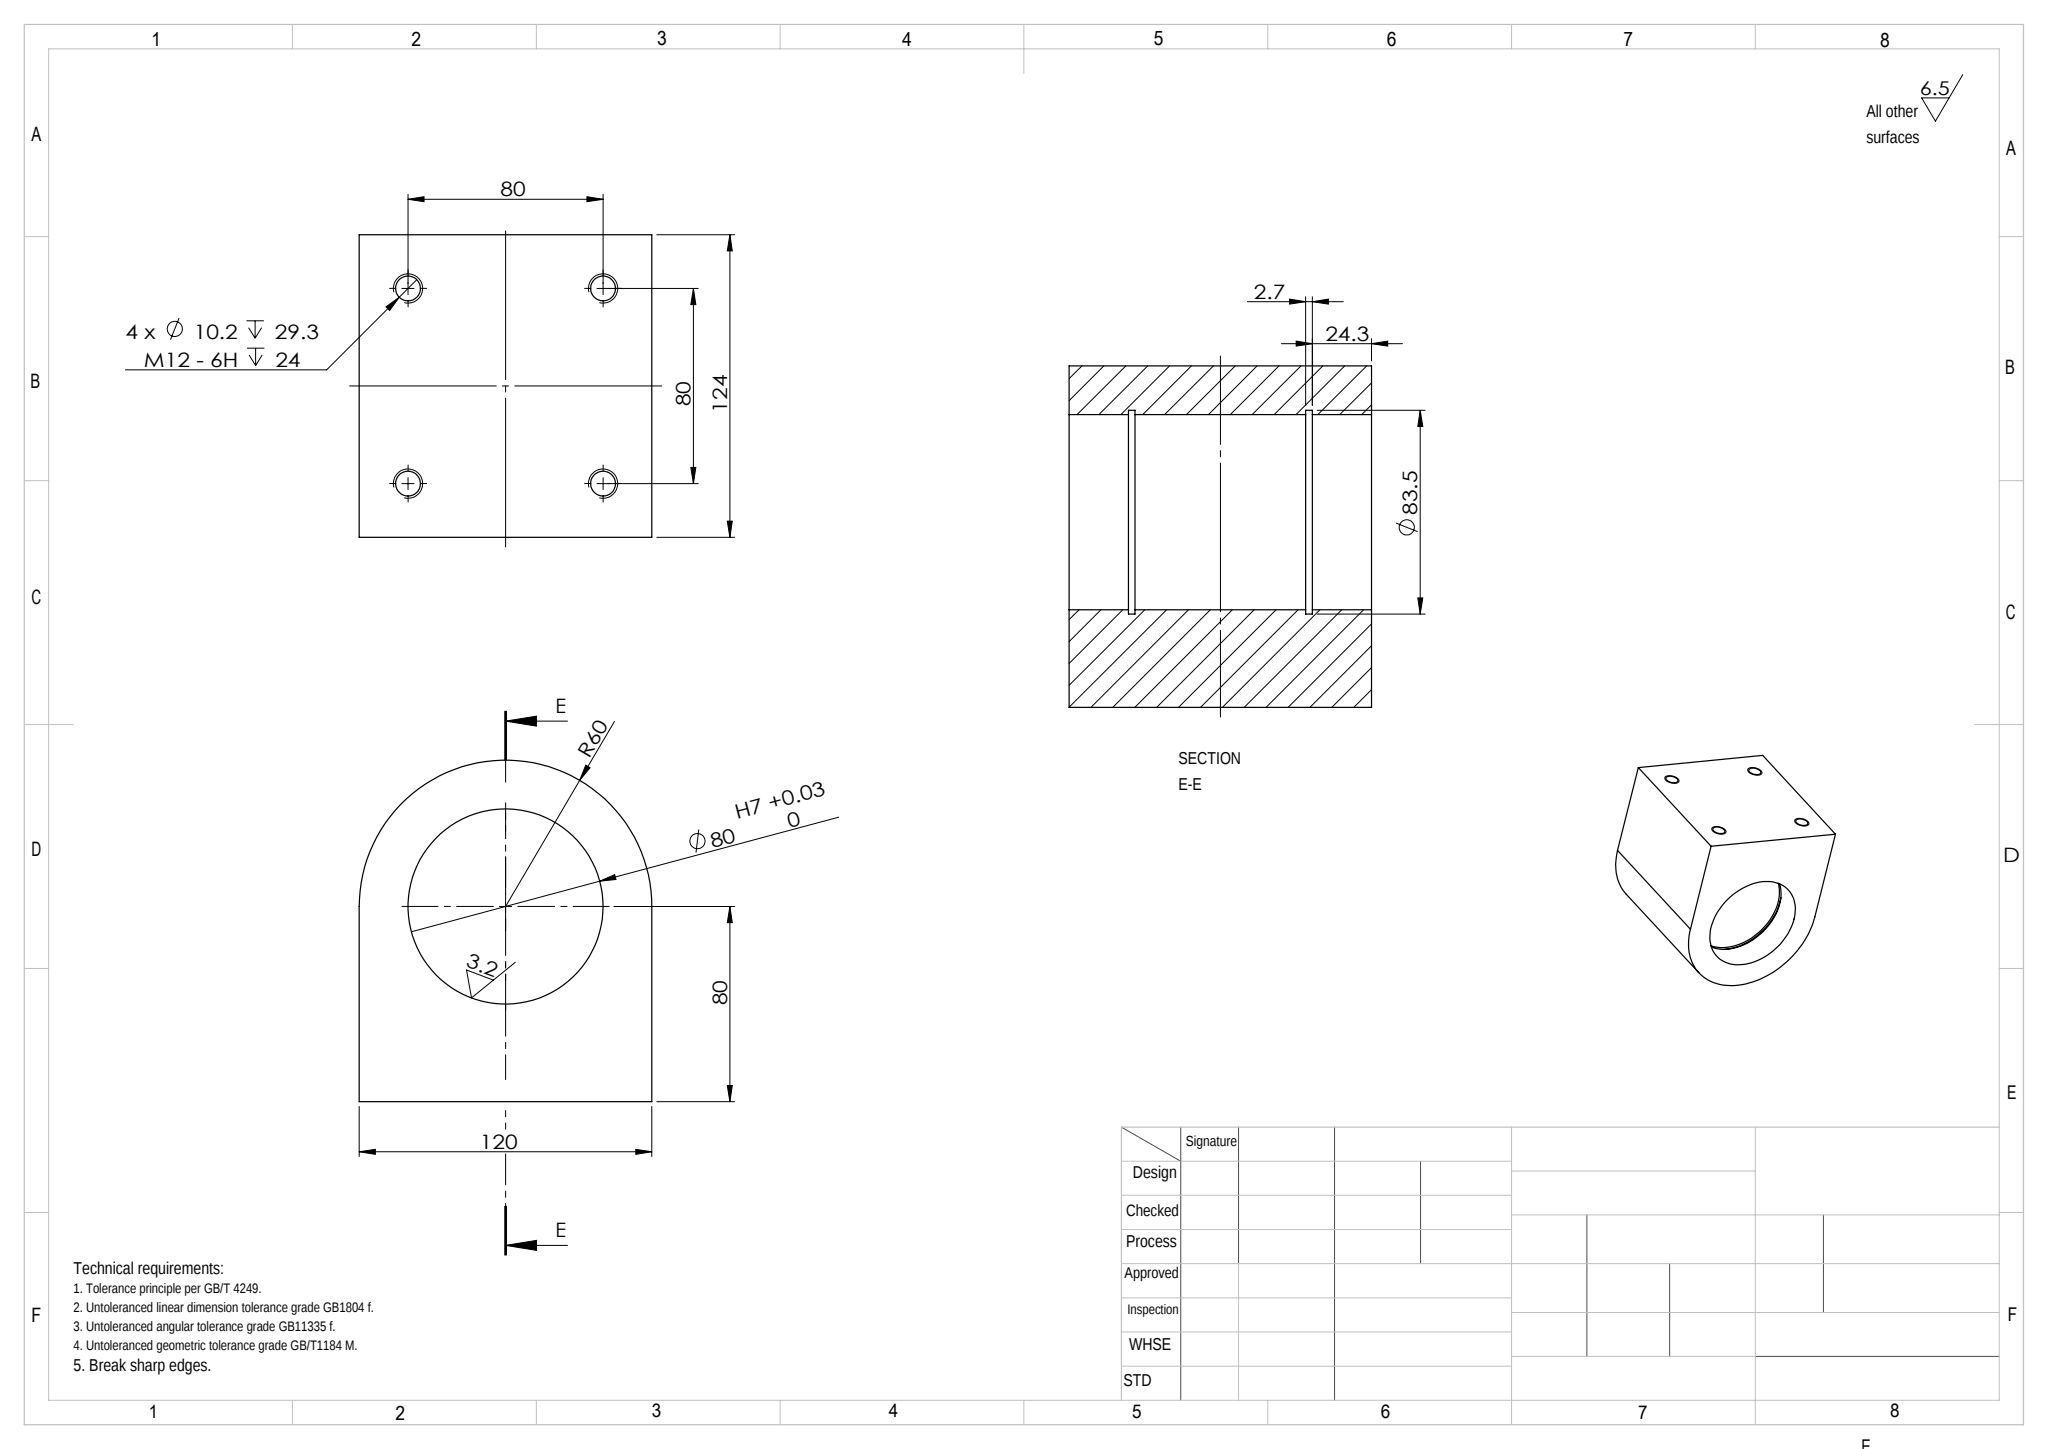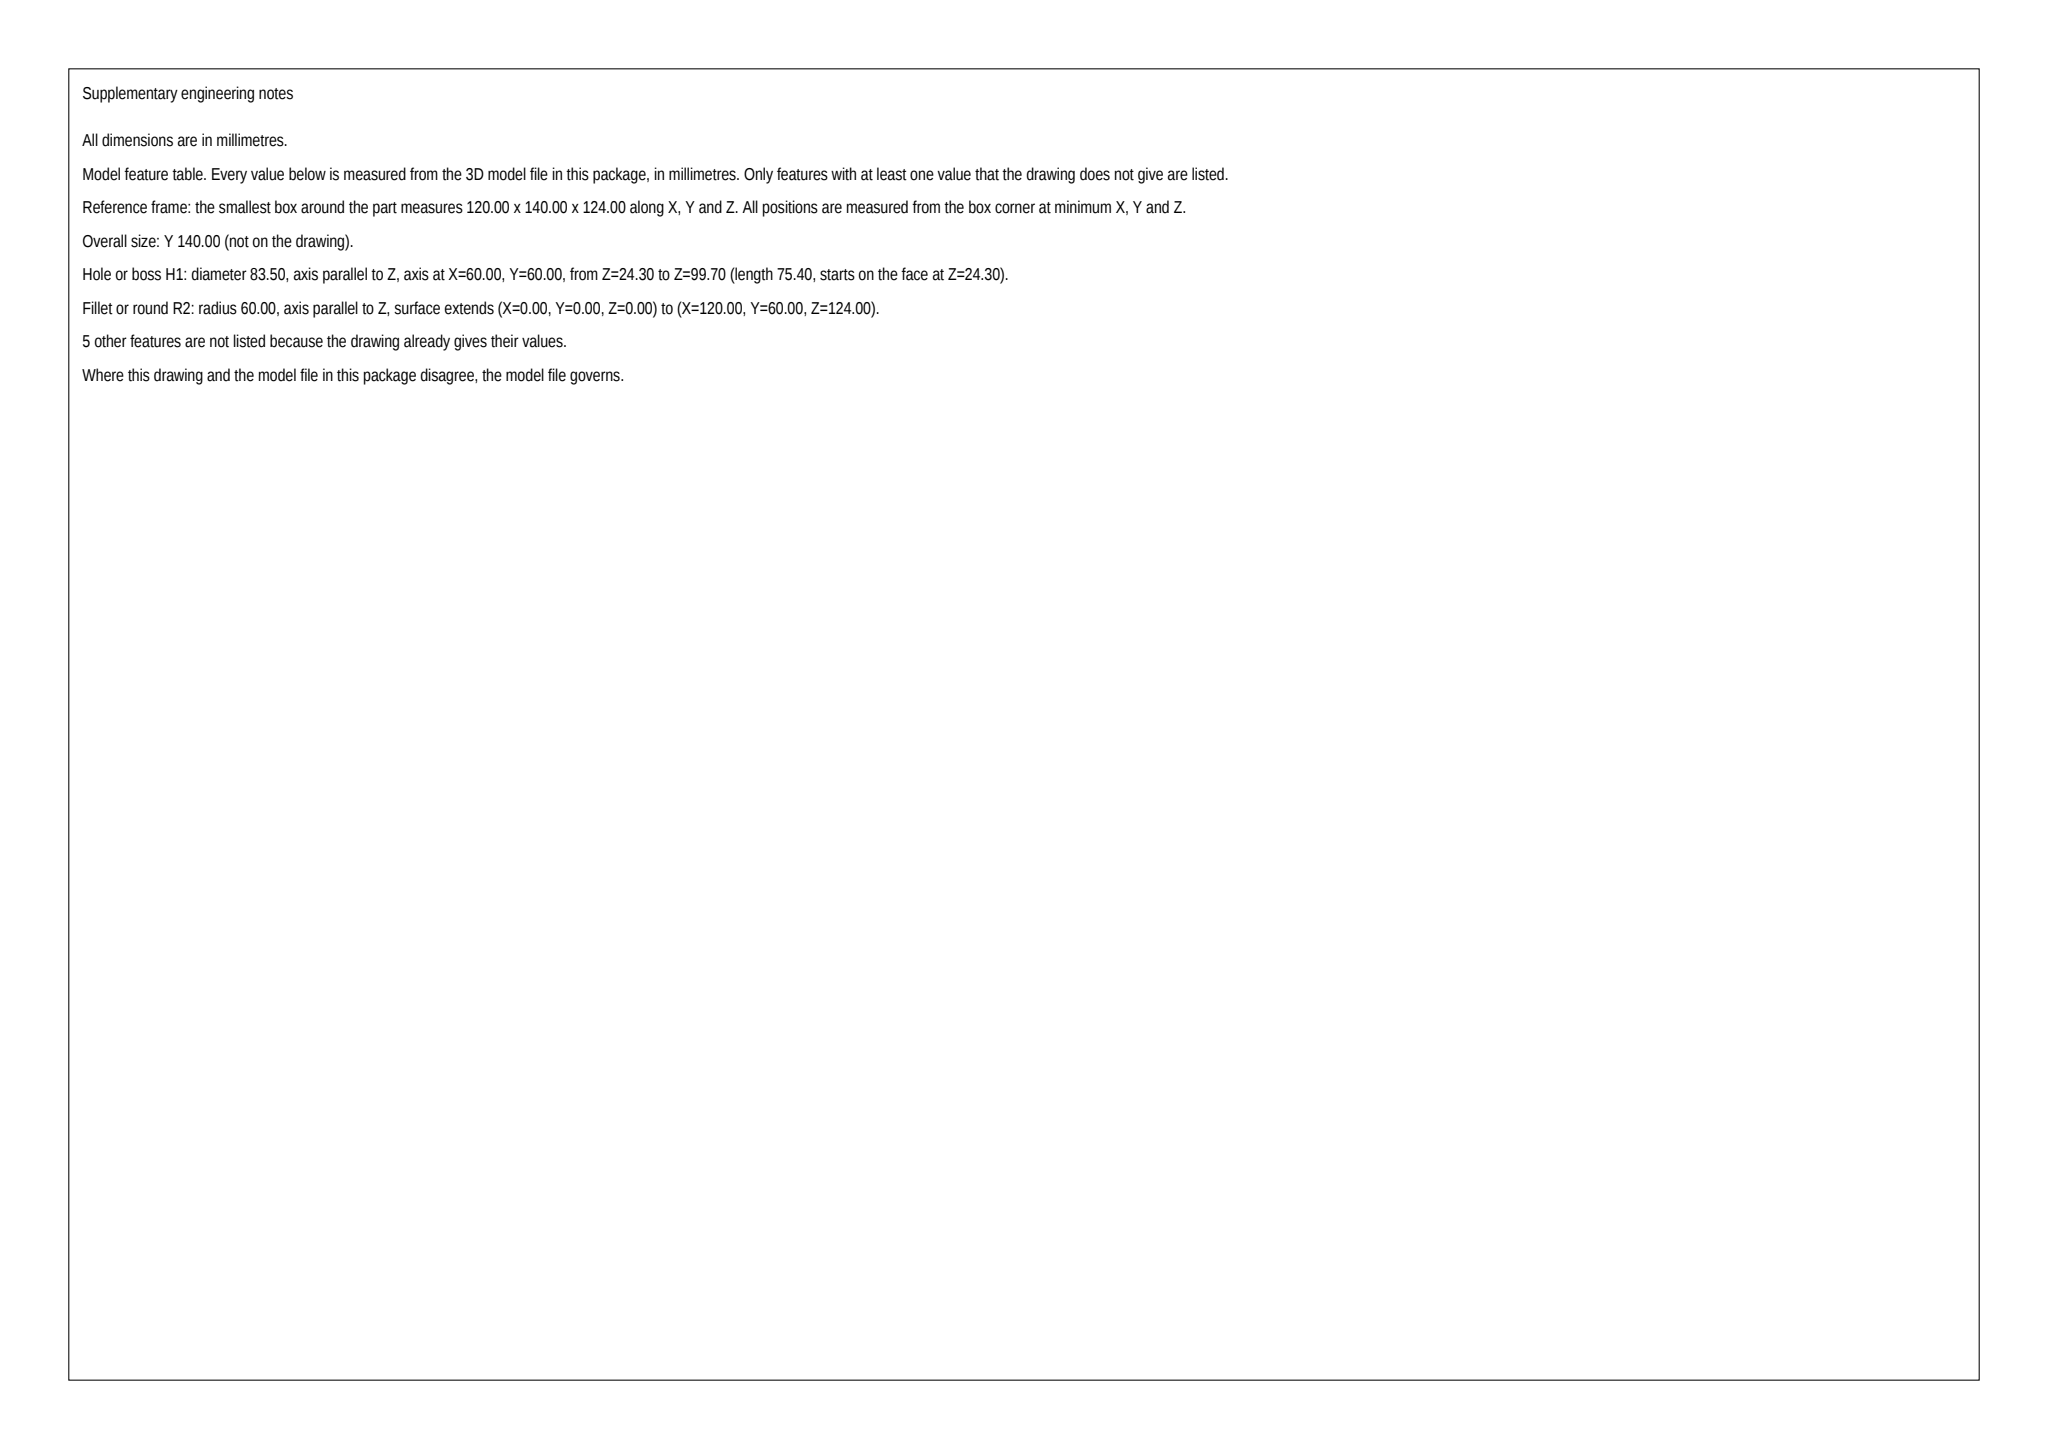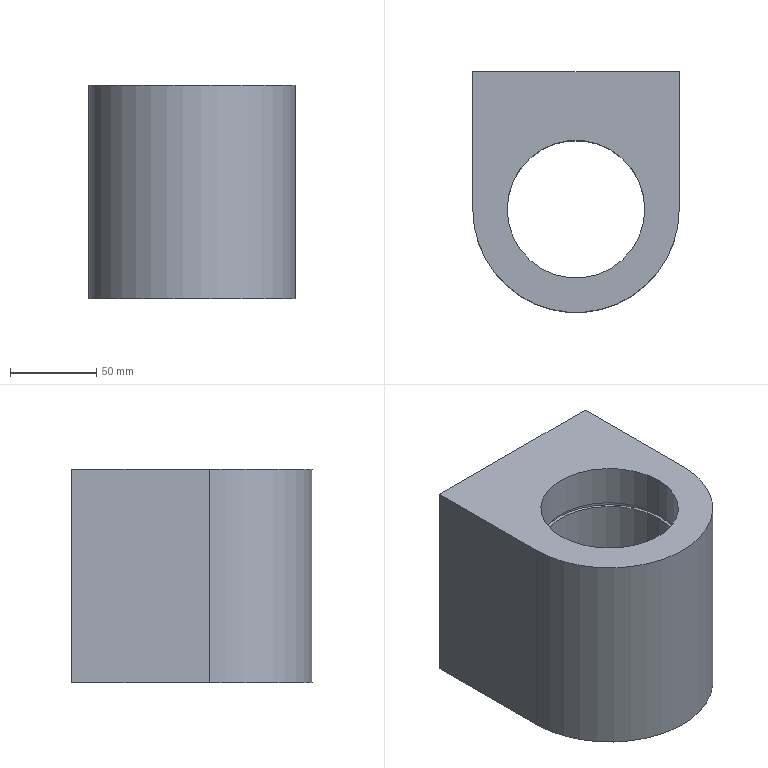Part | SolidWorks | mm | 1 solid | 36 faces | box 120 x 140 x 124 mm | volume 1255990 mm3 | cylinder 19 | plane 9 | cone 8 | commonest cylinder face diameters 10.2 x8 80 x6 83.5 x4 120 x1
Drawing notes:
2X GROOVE Ø83.5 x 2.7 WIDE IN Ø80 BORE, 24.3 FROM EACH END | from the solid: cyl dia 83.5 len 2.7 at z=24.3-27.0 and z=97.0-99.7; bore Ø80 len 124
2X GRV IN Ø80 BORE: Ø83.5 x 2.7 WIDE, 24.3 FROM EACH END | from the solid: cyl Ø83.5 axis z len 2.7 at z=24.3-27.0 and z=97.0-99.7; part length 124
build123d program:
from build123d import *

# Parameters (mm, degrees)
SKETCH1_R              = 60
SKETCH1_R_2            = 40
BOSS_EXTRUDE1_DEPTH    = 62
BOSS_EXTRUDE2_DEPTH    = 62
SKETCH3_R              = 41.75
SKETCH3_R_2            = 40
CUT_EXTRUDE1_DEPTH     = 2.7
M12_TAPPED_HOLE1_D     = 10.2
M12_TAPPED_HOLE1_DEPTH = 29.25
M12_TAPPED_HOLE1_TIP   = 3.064


with BuildPart() as part:
    # Sketch1 → Boss-Extrude1 (new, symmetric)
    with BuildSketch(Plane.XY):
        Circle(SKETCH1_R)
        Circle(SKETCH1_R_2, mode=Mode.SUBTRACT)
    extrude(amount=BOSS_EXTRUDE1_DEPTH, both=True)

    # Sketch2 → Boss-Extrude2 (add, symmetric)
    with BuildSketch(Plane.XY):
        with BuildLine():
            Line((40, 0), (60, 0))
            Line((60, 0), (60, 80))
            Line((60, 80), (-60, 80))
            Line((-60, 80), (-60, 0))
            Line((-60, 0), (-40, 0))
            ThreePointArc((-40, 0), (0, 40), (40, 0))
        make_face()
    extrude(amount=BOSS_EXTRUDE2_DEPTH, both=True)

    # Sketch3 → Cut-Extrude1 (cut)
    with BuildSketch(Plane(origin=(0, 0, -37.7), x_dir=(-1, 0, 0), z_dir=(0, 0, -1))):
        Circle(SKETCH3_R)
        Circle(SKETCH3_R_2, mode=Mode.SUBTRACT)
    cut_extrude1 = extrude(amount=-CUT_EXTRUDE1_DEPTH, mode=Mode.SUBTRACT)

    # Mirror1: Cut-Extrude1 across plane
    add(cut_extrude1.mirror(Plane.XY), mode=Mode.SUBTRACT)

    # M12 Tapped Hole1
    with Locations(Plane(origin=(-40, 80, 40), x_dir=(1, 0, 0), z_dir=(0, 1, 0))):
        with Locations((0, 0), (0, 80), (80, 80), (80, 0)):
            Hole(M12_TAPPED_HOLE1_D / 2, depth=M12_TAPPED_HOLE1_DEPTH)
            with Locations((0, 0, -(M12_TAPPED_HOLE1_DEPTH + M12_TAPPED_HOLE1_TIP / 2))):  # 118° drill point
                Cone(0, M12_TAPPED_HOLE1_D / 2, M12_TAPPED_HOLE1_TIP, mode=Mode.SUBTRACT)


solid = part.part